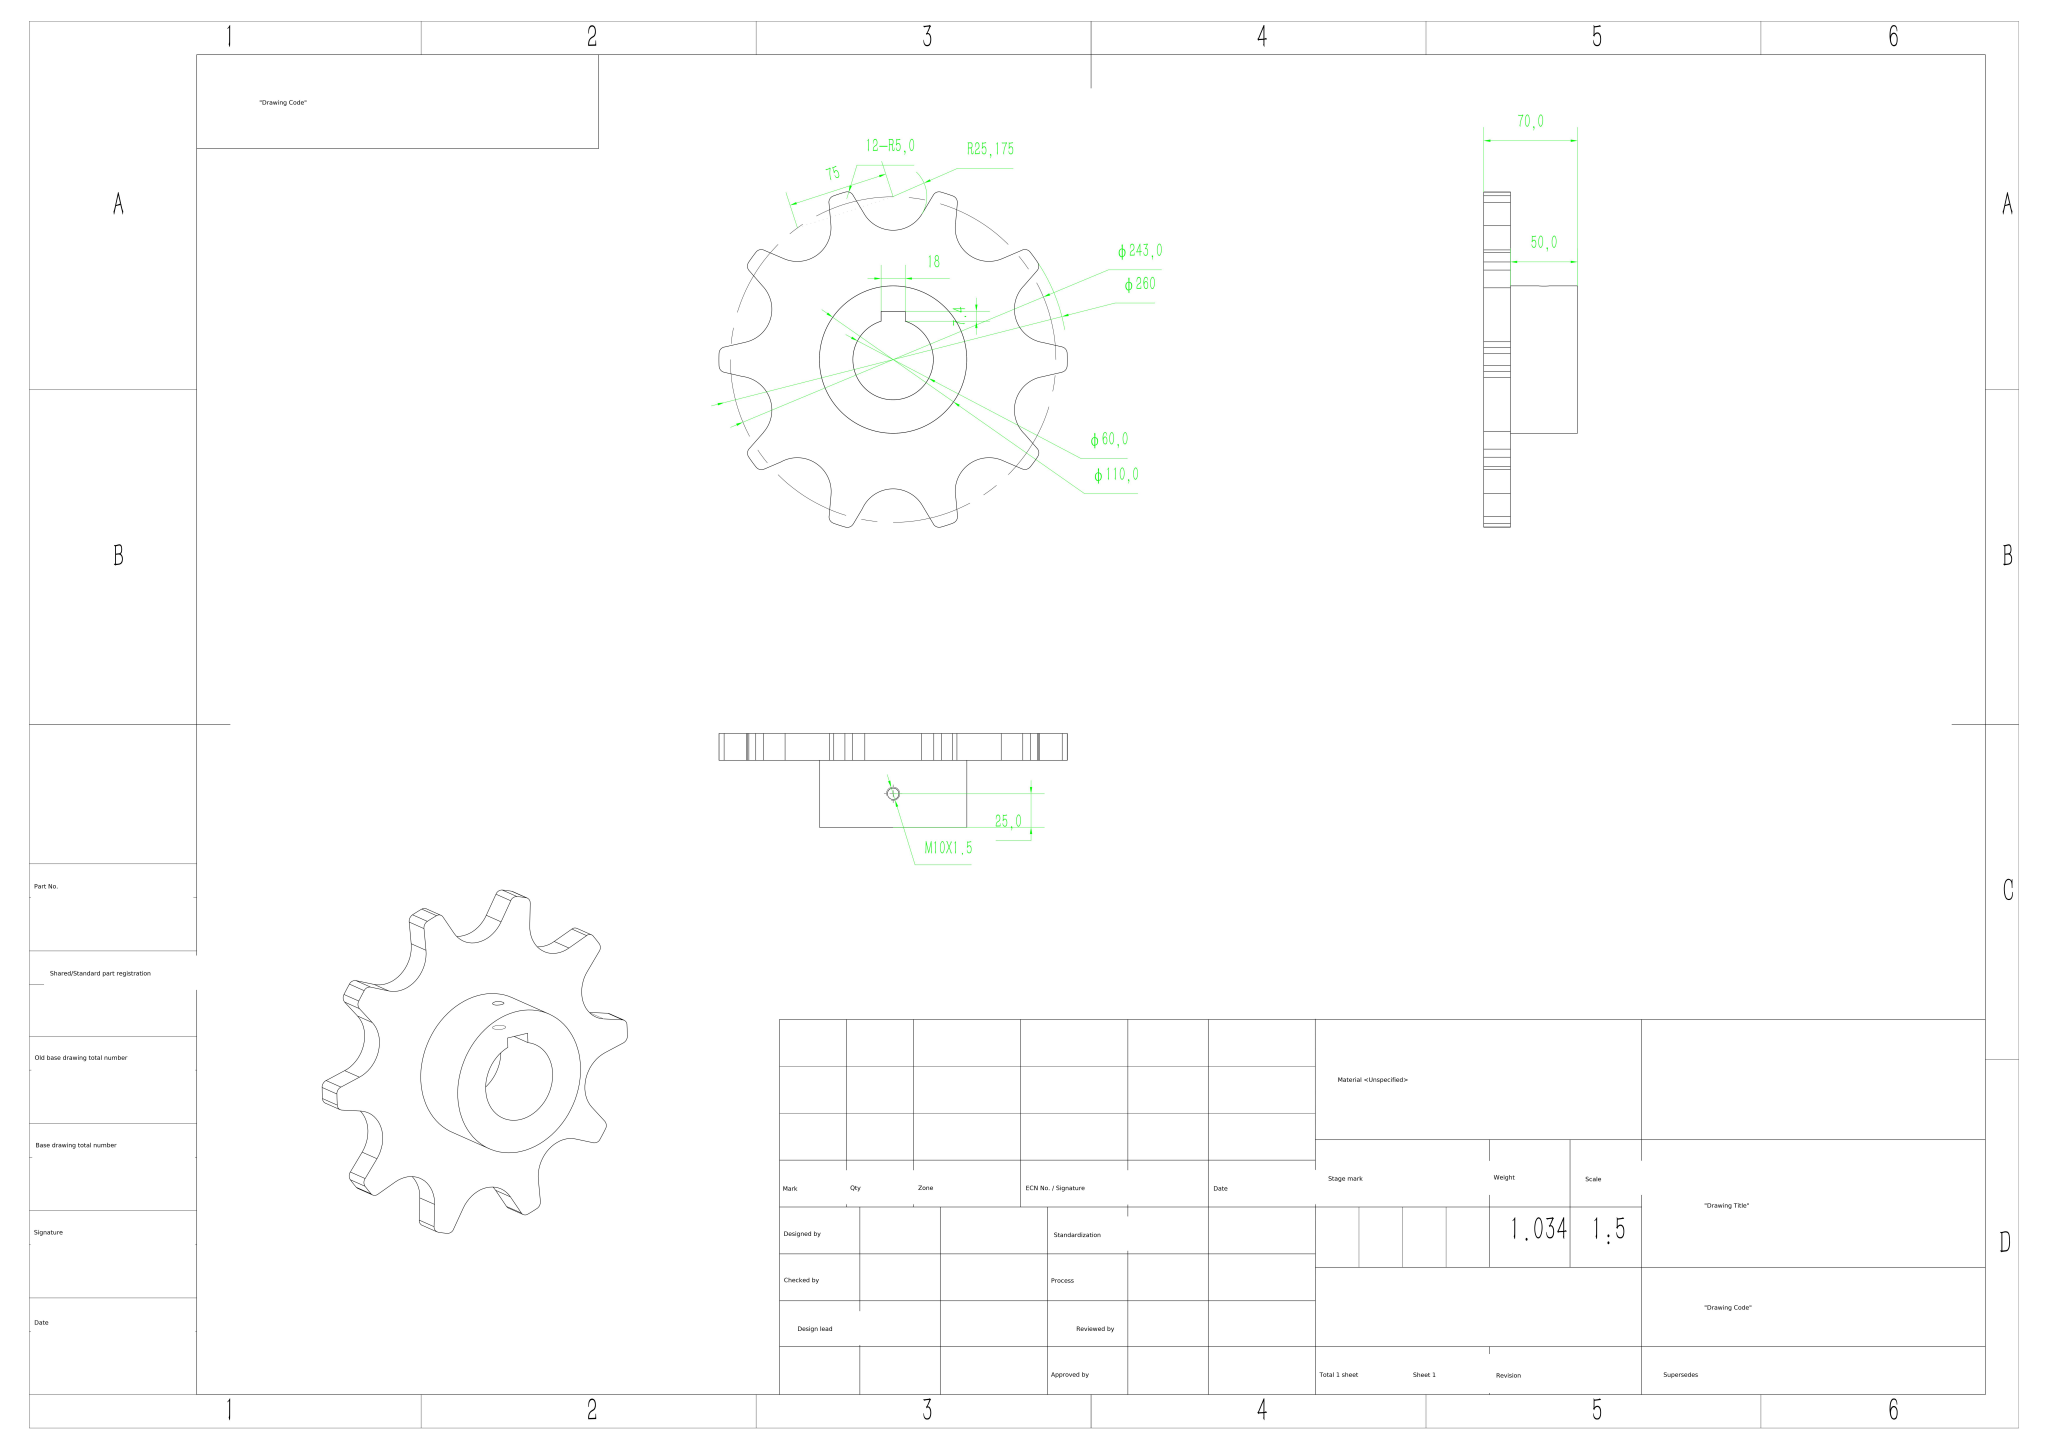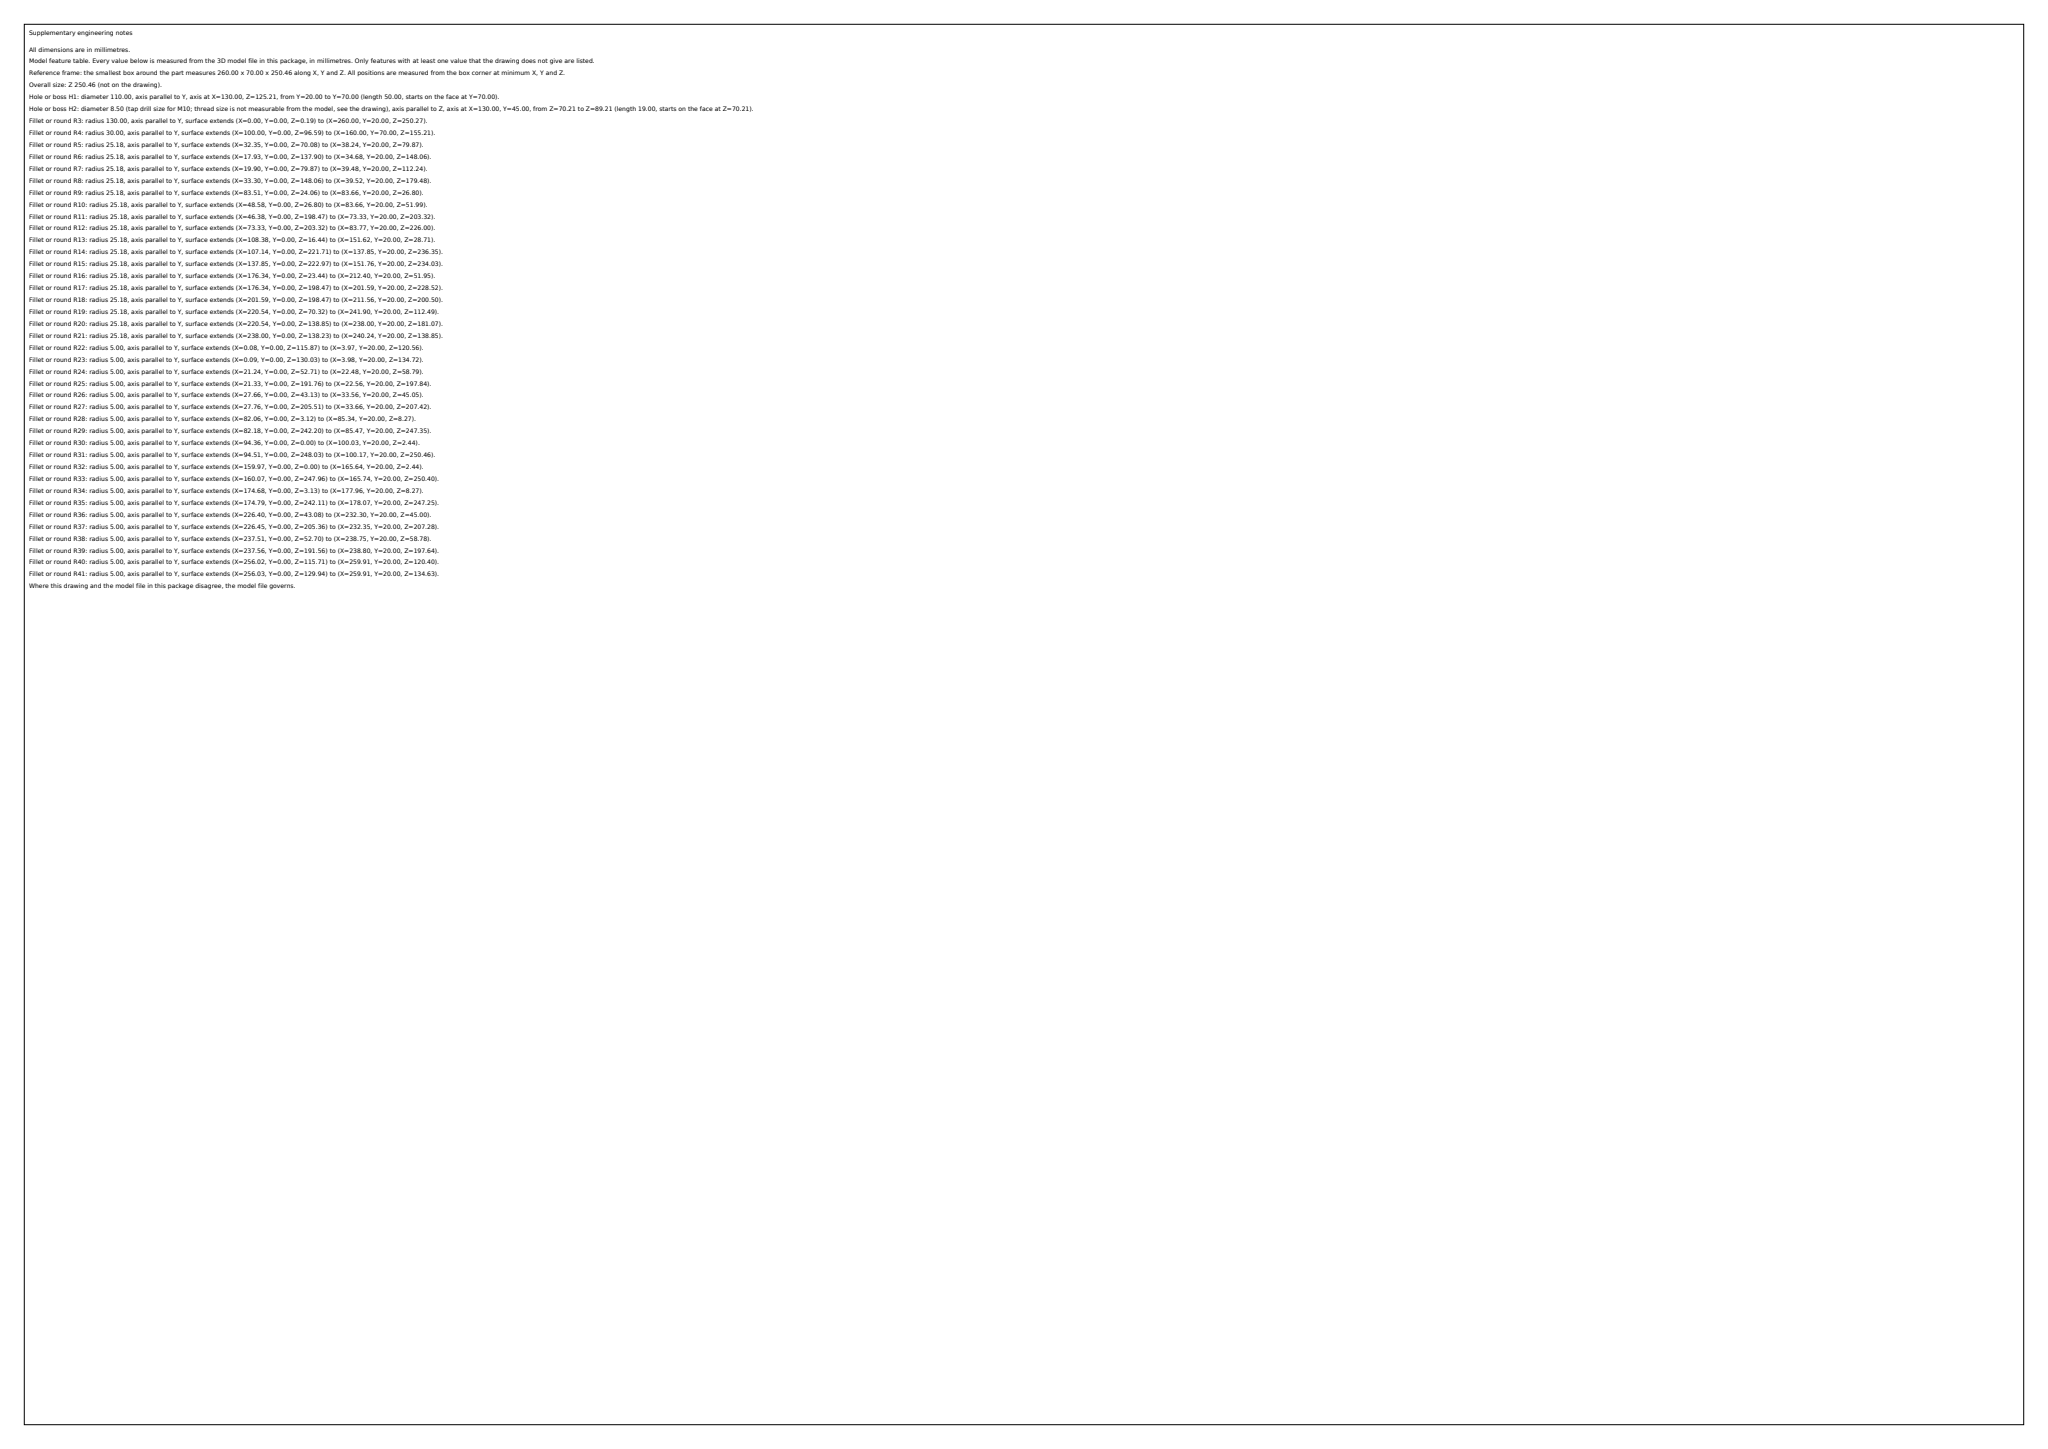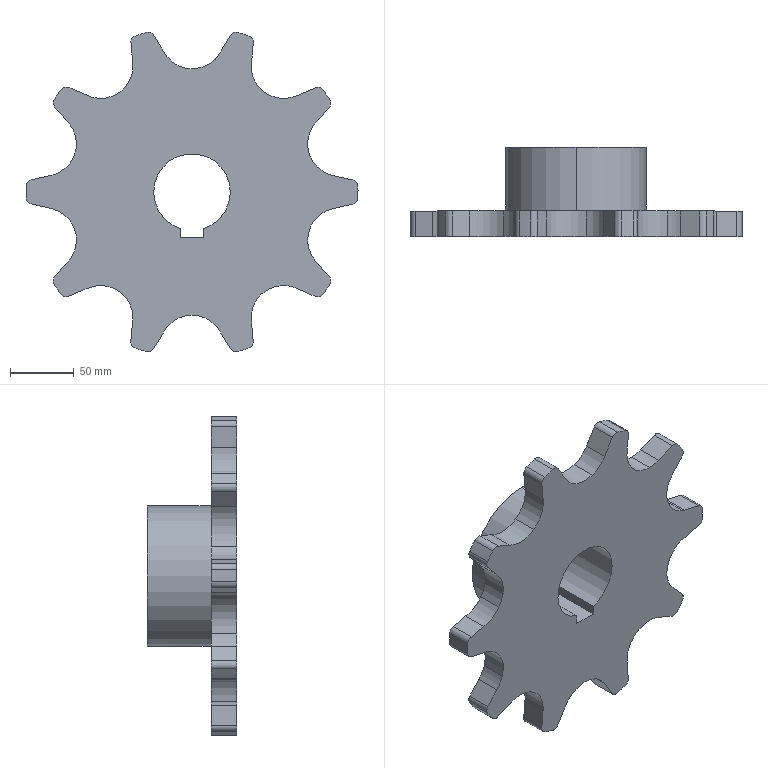Part | SolidWorks | mm | 1 solid | 85 faces | box 260 x 70 x 250.46 mm | volume 1034929 mm3 | cylinder 59 | plane 26 | commonest cylinder face diameters 10 x24 50.35 x20 260 x10 8.5 x2 110 x2 60 x1